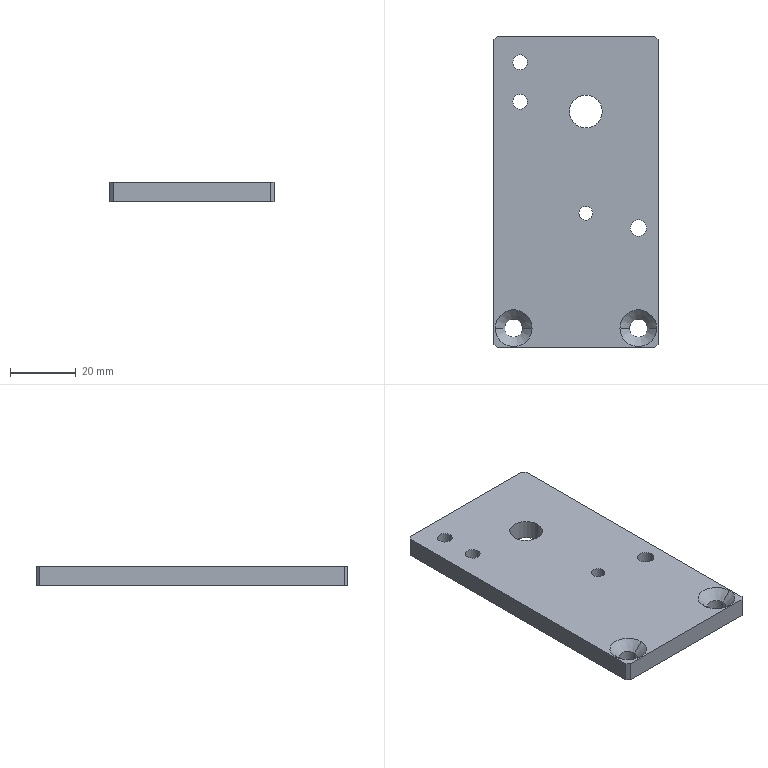Component | SolidWorks | JCT-03-02SmallUprightPlate-1 | 1 solid | 28 faces | box 50 x 95 x 6 mm | volume 27151 mm3 | cylinder 14 | plane 10 | cone 4 | commonest cylinder face diameters 4.5 x4 5.5 x4 10 x2 4.2 x2 5 x2
build123d program:
from build123d import *

# Parameters (mm, degrees)
SKETCH1_W                                            = 50
SKETCH1_H                                            = 95
EXTRUDE1_DEPTH                                       = 3
M5_HEXAGONAL_COUNTERSUNK_SCREW_COUNTERSU_D           = 5.5
M5_HEXAGONAL_COUNTERSUNK_SCREW_COUNTERSU_CSINK_D     = 11.2
M5_HEXAGONAL_COUNTERSUNK_SCREW_COUNTERSU_CSINK_ANGLE = 90
M5_TAPPED_HOLE1_D                                    = 5
M5_TAPPED_HOLE2_D                                    = 4.2
M10_TAPPED_HOLE1_D                                   = 10
SKETCH10_R                                           = 2.25
EXTRUDE2_DEPTH                                       = 108.522
CHAMFER1_SIZE                                        = 1


with BuildPart() as part:
    # Sketch1 → Extrude1 (new, symmetric)
    with BuildSketch(Plane(origin=(0, 0, 0), x_dir=(0, 0, -1), z_dir=(1, 0, 0))):
        with Locations((-25, 47.5)):
            Rectangle(SKETCH1_W, SKETCH1_H)
    extrude(amount=EXTRUDE1_DEPTH, both=True)

    # M5 Hexagonal Countersunk Screw Countersu (through all)
    with Locations(Plane(origin=(3, 0, 0), x_dir=(0, 0, -1), z_dir=(1, 0, 0))):
        with Locations((-44, 6), (-6, 6)):
            CounterSinkHole(M5_HEXAGONAL_COUNTERSUNK_SCREW_COUNTERSU_D / 2, M5_HEXAGONAL_COUNTERSUNK_SCREW_COUNTERSU_CSINK_D / 2, counter_sink_angle=M5_HEXAGONAL_COUNTERSUNK_SCREW_COUNTERSU_CSINK_ANGLE)

    # M5 Tapped Hole1 (through all)
    with Locations(Plane(origin=(3, 0, 0), x_dir=(0, 0, -1), z_dir=(1, 0, 0))):
        with Locations((-6, 36.5)):
            Hole(M5_TAPPED_HOLE1_D / 2)

    # M5 Tapped Hole2 (through all)
    with Locations(Plane(origin=(3, 0, 0), x_dir=(0, 0, -1), z_dir=(1, 0, 0))):
        with Locations((-22, 41)):
            Hole(M5_TAPPED_HOLE2_D / 2)

    # M10 Tapped Hole1 (through all)
    with Locations(Plane(origin=(3, 0, 0), x_dir=(0, 0, -1), z_dir=(1, 0, 0))):
        with Locations((-22, 72)):
            Hole(M10_TAPPED_HOLE1_D / 2)

    # Sketch10 → Extrude2 (cut, through all)
    with BuildSketch(Plane(origin=(3, 0, 0), x_dir=(0, 0, -1), z_dir=(1, 0, 0))):
        with Locations((-42, 87)):
            Circle(SKETCH10_R)
        with Locations((-42, 75)):
            Circle(SKETCH10_R)
    extrude(amount=-EXTRUDE2_DEPTH, mode=Mode.SUBTRACT)

    # Chamfer1
    chamfer1_edges = [part.edges().sort_by_distance(p)[0] for p in [
        (0, 0, 0),
        (0, 0, 50),
        (0, 95, 50),
        (0, 95, 0),
    ]]
    chamfer(chamfer1_edges, length=CHAMFER1_SIZE)


solid = part.part

# Placed as in the assembly
solid = solid.moved(Location((29.266, -2.701, 59), (0, -90, 0)))
STEP:
#1=CARTESIAN_POINT('',(-0.5899,2.846,2.205));
#2=VERTEX_POINT('',#1);
#3=CARTESIAN_POINT('',(-0.4127,2.846,2.205));
#4=VERTEX_POINT('',#3);
#5=CARTESIAN_POINT('',(-0.5013,2.846,2.205));
#6=DIRECTION('',(0.,-0.,1.));
#7=DIRECTION('',(1.,0.,0.));
#8=AXIS2_PLACEMENT_3D('',#5,#6,#7);
#9=CIRCLE('',#8,0.08858);
#10=EDGE_CURVE('',#2,#4,#9,.T.);
#11=ORIENTED_EDGE('',*,*,#10,.F.);
#12=CARTESIAN_POINT('',(-0.5899,2.846,2.441));
#13=VERTEX_POINT('',#12);
#14=CARTESIAN_POINT('',(-0.5899,2.846,2.205));
#15=DIRECTION('',(0.,-0.,1.));
#16=VECTOR('',#15,39.37);
#17=LINE('',#14,#16);
#18=EDGE_CURVE('',#2,#13,#17,.T.);
#19=ORIENTED_EDGE('',*,*,#18,.T.);
#20=CARTESIAN_POINT('',(-0.4127,2.846,2.441));
#21=VERTEX_POINT('',#20);
#22=CARTESIAN_POINT('',(-0.5013,2.846,2.441));
#23=DIRECTION('',(0.,-0.,1.));
#24=DIRECTION('',(1.,0.,0.));
#25=AXIS2_PLACEMENT_3D('',#22,#23,#24);
#26=CIRCLE('',#25,0.08858);
#27=EDGE_CURVE('',#13,#21,#26,.T.);
#28=ORIENTED_EDGE('',*,*,#27,.T.);
#29=CARTESIAN_POINT('',(-0.4127,2.846,2.205));
#30=DIRECTION('',(0.,-0.,1.));
#31=VECTOR('',#30,39.37);
#32=LINE('',#29,#31);
#33=EDGE_CURVE('',#4,#21,#32,.T.);
#34=ORIENTED_EDGE('',*,*,#33,.F.);
#35=EDGE_LOOP('',(#11,#19,#28,#34));
#36=FACE_OUTER_BOUND('',#35,.T.);
#37=CARTESIAN_POINT('',(-0.5013,2.846,2.205));
#38=DIRECTION('',(0.,-0.,1.));
#39=DIRECTION('',(1.,0.,0.));
#40=AXIS2_PLACEMENT_3D('',#37,#38,#39);
#41=CYLINDRICAL_SURFACE('',#40,0.08858);
#42=ADVANCED_FACE('',(#36),#41,.F.);
#43=CARTESIAN_POINT('',(-0.5899,3.319,2.205));
#44=VERTEX_POINT('',#43);
#45=CARTESIAN_POINT('',(-0.4127,3.319,2.205));
#46=VERTEX_POINT('',#45);
#47=CARTESIAN_POINT('',(-0.5013,3.319,2.205));
#48=DIRECTION('',(0.,-0.,1.));
#49=DIRECTION('',(1.,0.,0.));
#50=AXIS2_PLACEMENT_3D('',#47,#48,#49);
#51=CIRCLE('',#50,0.08858);
#52=EDGE_CURVE('',#44,#46,#51,.T.);
#53=ORIENTED_EDGE('',*,*,#52,.F.);
#54=CARTESIAN_POINT('',(-0.5899,3.319,2.441));
#55=VERTEX_POINT('',#54);
#56=CARTESIAN_POINT('',(-0.5899,3.319,2.205));
#57=DIRECTION('',(0.,-0.,1.));
#58=VECTOR('',#57,39.37);
#59=LINE('',#56,#58);
#60=EDGE_CURVE('',#44,#55,#59,.T.);
#61=ORIENTED_EDGE('',*,*,#60,.T.);
#62=CARTESIAN_POINT('',(-0.4127,3.319,2.441));
#63=VERTEX_POINT('',#62);
#64=CARTESIAN_POINT('',(-0.5013,3.319,2.441));
#65=DIRECTION('',(0.,-0.,1.));
#66=DIRECTION('',(1.,0.,0.));
#67=AXIS2_PLACEMENT_3D('',#64,#65,#66);
#68=CIRCLE('',#67,0.08858);
#69=EDGE_CURVE('',#55,#63,#68,.T.);
#70=ORIENTED_EDGE('',*,*,#69,.T.);
#71=CARTESIAN_POINT('',(-0.4127,3.319,2.205));
#72=DIRECTION('',(0.,-0.,1.));
#73=VECTOR('',#72,39.37);
#74=LINE('',#71,#73);
#75=EDGE_CURVE('',#46,#63,#74,.T.);
#76=ORIENTED_EDGE('',*,*,#75,.F.);
#77=EDGE_LOOP('',(#53,#61,#70,#76));
#78=FACE_OUTER_BOUND('',#77,.T.);
#79=CARTESIAN_POINT('',(-0.5013,3.319,2.205));
#80=DIRECTION('',(0.,-0.,1.));
#81=DIRECTION('',(1.,0.,0.));
#82=AXIS2_PLACEMENT_3D('',#79,#80,#81);
#83=CYLINDRICAL_SURFACE('',#82,0.08858);
#84=ADVANCED_FACE('',(#78),#83,.F.);
#85=CARTESIAN_POINT('',(0.08922,2.728,2.205));
#86=VERTEX_POINT('',#85);
#87=CARTESIAN_POINT('',(0.4829,2.728,2.205));
#88=VERTEX_POINT('',#87);
#89=CARTESIAN_POINT('',(0.2861,2.728,2.205));
#90=DIRECTION('',(0.,-0.,1.));
#91=DIRECTION('',(1.,0.,0.));
#92=AXIS2_PLACEMENT_3D('',#89,#90,#91);
#93=CIRCLE('',#92,0.1969);
#94=EDGE_CURVE('',#86,#88,#93,.T.);
#95=ORIENTED_EDGE('',*,*,#94,.F.);
#96=CARTESIAN_POINT('',(0.08922,2.728,2.441));
#97=VERTEX_POINT('',#96);
#98=CARTESIAN_POINT('',(0.08922,2.728,2.441));
#99=DIRECTION('',(0.,-0.,1.));
#100=VECTOR('',#99,39.37);
#101=LINE('',#98,#100);
#102=EDGE_CURVE('',#86,#97,#101,.T.);
#103=ORIENTED_EDGE('',*,*,#102,.T.);
#104=CARTESIAN_POINT('',(0.4829,2.728,2.441));
#105=VERTEX_POINT('',#104);
#106=CARTESIAN_POINT('',(0.2861,2.728,2.441));
#107=DIRECTION('',(0.,-0.,1.));
#108=DIRECTION('',(1.,0.,0.));
#109=AXIS2_PLACEMENT_3D('',#106,#107,#108);
#110=CIRCLE('',#109,0.1969);
#111=EDGE_CURVE('',#97,#105,#110,.T.);
#112=ORIENTED_EDGE('',*,*,#111,.T.);
#113=CARTESIAN_POINT('',(0.4829,2.728,2.441));
#114=DIRECTION('',(0.,-0.,1.));
#115=VECTOR('',#114,39.37);
#116=LINE('',#113,#115);
#117=EDGE_CURVE('',#88,#105,#116,.T.);
#118=ORIENTED_EDGE('',*,*,#117,.F.);
#119=EDGE_LOOP('',(#95,#103,#112,#118));
#120=FACE_OUTER_BOUND('',#119,.T.);
#121=CARTESIAN_POINT('',(0.2861,2.728,2.441));
#122=DIRECTION('',(0.,-0.,1.));
#123=DIRECTION('',(1.,0.,0.));
#124=AXIS2_PLACEMENT_3D('',#121,#122,#123);
#125=CYLINDRICAL_SURFACE('',#124,0.1969);
#126=ADVANCED_FACE('',(#120),#125,.F.);
#127=CARTESIAN_POINT('',(0.2034,1.508,2.205));
#128=VERTEX_POINT('',#127);
#129=CARTESIAN_POINT('',(0.3688,1.508,2.205));
#130=VERTEX_POINT('',#129);
#131=CARTESIAN_POINT('',(0.2861,1.508,2.205));
#132=DIRECTION('',(0.,-0.,1.));
#133=DIRECTION('',(1.,0.,0.));
#134=AXIS2_PLACEMENT_3D('',#131,#132,#133);
#135=CIRCLE('',#134,0.08268);
#136=EDGE_CURVE('',#128,#130,#135,.T.);
#137=ORIENTED_EDGE('',*,*,#136,.F.);
#138=CARTESIAN_POINT('',(0.2034,1.508,2.441));
#139=VERTEX_POINT('',#138);
#140=CARTESIAN_POINT('',(0.2034,1.508,2.441));
#141=DIRECTION('',(0.,-0.,1.));
#142=VECTOR('',#141,39.37);
#143=LINE('',#140,#142);
#144=EDGE_CURVE('',#128,#139,#143,.T.);
#145=ORIENTED_EDGE('',*,*,#144,.T.);
#146=CARTESIAN_POINT('',(0.3688,1.508,2.441));
#147=VERTEX_POINT('',#146);
#148=CARTESIAN_POINT('',(0.2861,1.508,2.441));
#149=DIRECTION('',(0.,-0.,1.));
#150=DIRECTION('',(1.,0.,0.));
#151=AXIS2_PLACEMENT_3D('',#148,#149,#150);
#152=CIRCLE('',#151,0.08268);
#153=EDGE_CURVE('',#139,#147,#152,.T.);
#154=ORIENTED_EDGE('',*,*,#153,.T.);
#155=CARTESIAN_POINT('',(0.3688,1.508,2.441));
#156=DIRECTION('',(0.,-0.,1.));
#157=VECTOR('',#156,39.37);
#158=LINE('',#155,#157);
#159=EDGE_CURVE('',#130,#147,#158,.T.);
#160=ORIENTED_EDGE('',*,*,#159,.F.);
#161=EDGE_LOOP('',(#137,#145,#154,#160));
#162=FACE_OUTER_BOUND('',#161,.T.);
#163=CARTESIAN_POINT('',(0.2861,1.508,2.441));
#164=DIRECTION('',(0.,-0.,1.));
#165=DIRECTION('',(1.,0.,0.));
#166=AXIS2_PLACEMENT_3D('',#163,#164,#165);
#167=CYLINDRICAL_SURFACE('',#166,0.08268);
#168=ADVANCED_FACE('',(#162),#167,.F.);
#169=CARTESIAN_POINT('',(0.8176,1.331,2.205));
#170=VERTEX_POINT('',#169);
#171=CARTESIAN_POINT('',(1.014,1.331,2.205));
#172=VERTEX_POINT('',#171);
#173=CARTESIAN_POINT('',(0.916,1.331,2.205));
#174=DIRECTION('',(0.,-0.,1.));
#175=DIRECTION('',(1.,0.,0.));
#176=AXIS2_PLACEMENT_3D('',#173,#174,#175);
#177=CIRCLE('',#176,0.09843);
#178=EDGE_CURVE('',#170,#172,#177,.T.);
#179=ORIENTED_EDGE('',*,*,#178,.F.);
#180=CARTESIAN_POINT('',(0.8176,1.331,2.441));
#181=VERTEX_POINT('',#180);
#182=CARTESIAN_POINT('',(0.8176,1.331,2.441));
#183=DIRECTION('',(0.,-0.,1.));
#184=VECTOR('',#183,39.37);
#185=LINE('',#182,#184);
#186=EDGE_CURVE('',#170,#181,#185,.T.);
#187=ORIENTED_EDGE('',*,*,#186,.T.);
#188=CARTESIAN_POINT('',(1.014,1.331,2.441));
#189=VERTEX_POINT('',#188);
#190=CARTESIAN_POINT('',(0.916,1.331,2.441));
#191=DIRECTION('',(0.,-0.,1.));
#192=DIRECTION('',(1.,0.,0.));
#193=AXIS2_PLACEMENT_3D('',#190,#191,#192);
#194=CIRCLE('',#193,0.09843);
#195=EDGE_CURVE('',#181,#189,#194,.T.);
#196=ORIENTED_EDGE('',*,*,#195,.T.);
#197=CARTESIAN_POINT('',(1.014,1.331,2.441));
#198=DIRECTION('',(0.,-0.,1.));
#199=VECTOR('',#198,39.37);
#200=LINE('',#197,#199);
#201=EDGE_CURVE('',#172,#189,#200,.T.);
#202=ORIENTED_EDGE('',*,*,#201,.F.);
#203=EDGE_LOOP('',(#179,#187,#196,#202));
#204=FACE_OUTER_BOUND('',#203,.T.);
#205=CARTESIAN_POINT('',(0.916,1.331,2.441));
#206=DIRECTION('',(0.,-0.,1.));
#207=DIRECTION('',(1.,0.,0.));
#208=AXIS2_PLACEMENT_3D('',#205,#206,#207);
#209=CYLINDRICAL_SURFACE('',#208,0.09843);
#210=ADVANCED_FACE('',(#204),#209,.F.);
#211=CARTESIAN_POINT('',(-0.6883,0.1299,2.329));
#212=VERTEX_POINT('',#211);
#213=CARTESIAN_POINT('',(-0.4718,0.1299,2.329));
#214=VERTEX_POINT('',#213);
#215=CARTESIAN_POINT('',(-0.5801,0.1299,2.329));
#216=DIRECTION('',(0.,-0.,1.));
#217=DIRECTION('',(1.,-0.,0.));
#218=AXIS2_PLACEMENT_3D('',#215,#216,#217);
#219=CIRCLE('',#218,0.1083);
#220=EDGE_CURVE('',#212,#214,#219,.T.);
#221=ORIENTED_EDGE('',*,*,#220,.F.);
#222=CARTESIAN_POINT('',(-0.8005,0.1299,2.441));
#223=VERTEX_POINT('',#222);
#224=CARTESIAN_POINT('',(-0.8005,0.1299,2.441));
#225=DIRECTION('',(-0.7071,0.,0.7071));
#226=VECTOR('',#225,39.37);
#227=LINE('',#224,#226);
#228=EDGE_CURVE('',#212,#223,#227,.T.);
#229=ORIENTED_EDGE('',*,*,#228,.T.);
#230=CARTESIAN_POINT('',(-0.3596,0.1299,2.441));
#231=VERTEX_POINT('',#230);
#232=CARTESIAN_POINT('',(-0.5801,0.1299,2.441));
#233=DIRECTION('',(0.,-0.,1.));
#234=DIRECTION('',(1.,-0.,0.));
#235=AXIS2_PLACEMENT_3D('',#232,#233,#234);
#236=CIRCLE('',#235,0.2205);
#237=EDGE_CURVE('',#223,#231,#236,.T.);
#238=ORIENTED_EDGE('',*,*,#237,.T.);
#239=CARTESIAN_POINT('',(-0.3596,0.1299,2.441));
#240=DIRECTION('',(0.7071,-0.,0.7071));
#241=VECTOR('',#240,39.37);
#242=LINE('',#239,#241);
#243=EDGE_CURVE('',#214,#231,#242,.T.);
#244=ORIENTED_EDGE('',*,*,#243,.F.);
#245=EDGE_LOOP('',(#221,#229,#238,#244));
#246=FACE_OUTER_BOUND('',#245,.T.);
#247=CARTESIAN_POINT('',(-0.5801,0.1299,2.441));
#248=DIRECTION('',(0.,-0.,1.));
#249=DIRECTION('',(1.,-0.,0.));
#250=AXIS2_PLACEMENT_3D('',#247,#248,#249);
#251=CONICAL_SURFACE('',#250,0.2205,0.7854);
#252=ADVANCED_FACE('',(#246),#251,.F.);
#253=CARTESIAN_POINT('',(-0.6883,0.1299,2.205));
#254=VERTEX_POINT('',#253);
#255=CARTESIAN_POINT('',(-0.4718,0.1299,2.205));
#256=VERTEX_POINT('',#255);
#257=CARTESIAN_POINT('',(-0.5801,0.1299,2.205));
#258=DIRECTION('',(0.,-0.,1.));
#259=DIRECTION('',(1.,-0.,0.));
#260=AXIS2_PLACEMENT_3D('',#257,#258,#259);
#261=CIRCLE('',#260,0.1083);
#262=EDGE_CURVE('',#254,#256,#261,.T.);
#263=ORIENTED_EDGE('',*,*,#262,.F.);
#264=CARTESIAN_POINT('',(-0.6883,0.1299,2.441));
#265=DIRECTION('',(0.,-0.,1.));
#266=VECTOR('',#265,39.37);
#267=LINE('',#264,#266);
#268=EDGE_CURVE('',#254,#212,#267,.T.);
#269=ORIENTED_EDGE('',*,*,#268,.T.);
#270=ORIENTED_EDGE('',*,*,#220,.T.);
#271=CARTESIAN_POINT('',(-0.4718,0.1299,2.441));
#272=DIRECTION('',(0.,-0.,1.));
#273=VECTOR('',#272,39.37);
#274=LINE('',#271,#273);
#275=EDGE_CURVE('',#256,#214,#274,.T.);
#276=ORIENTED_EDGE('',*,*,#275,.F.);
#277=EDGE_LOOP('',(#263,#269,#270,#276));
#278=FACE_OUTER_BOUND('',#277,.T.);
#279=CARTESIAN_POINT('',(-0.5801,0.1299,2.441));
#280=DIRECTION('',(0.,-0.,1.));
#281=DIRECTION('',(1.,-0.,0.));
#282=AXIS2_PLACEMENT_3D('',#279,#280,#281);
#283=CYLINDRICAL_SURFACE('',#282,0.1083);
#284=ADVANCED_FACE('',(#278),#283,.F.);
#285=CARTESIAN_POINT('',(0.8077,0.1299,2.329));
#286=VERTEX_POINT('',#285);
#287=CARTESIAN_POINT('',(1.024,0.1299,2.329));
#288=VERTEX_POINT('',#287);
#289=CARTESIAN_POINT('',(0.916,0.1299,2.329));
#290=DIRECTION('',(0.,-0.,1.));
#291=DIRECTION('',(1.,-0.,0.));
#292=AXIS2_PLACEMENT_3D('',#289,#290,#291);
#293=CIRCLE('',#292,0.1083);
#294=EDGE_CURVE('',#286,#288,#293,.T.);
#295=ORIENTED_EDGE('',*,*,#294,.F.);
#296=CARTESIAN_POINT('',(0.6955,0.1299,2.441));
#297=VERTEX_POINT('',#296);
#298=CARTESIAN_POINT('',(0.6955,0.1299,2.441));
#299=DIRECTION('',(-0.7071,0.,0.7071));
#300=VECTOR('',#299,39.37);
#301=LINE('',#298,#300);
#302=EDGE_CURVE('',#286,#297,#301,.T.);
#303=ORIENTED_EDGE('',*,*,#302,.T.);
#304=CARTESIAN_POINT('',(1.136,0.1299,2.441));
#305=VERTEX_POINT('',#304);
#306=CARTESIAN_POINT('',(0.916,0.1299,2.441));
#307=DIRECTION('',(0.,-0.,1.));
#308=DIRECTION('',(1.,-0.,0.));
#309=AXIS2_PLACEMENT_3D('',#306,#307,#308);
#310=CIRCLE('',#309,0.2205);
#311=EDGE_CURVE('',#297,#305,#310,.T.);
#312=ORIENTED_EDGE('',*,*,#311,.T.);
#313=CARTESIAN_POINT('',(1.136,0.1299,2.441));
#314=DIRECTION('',(0.7071,-0.,0.7071));
#315=VECTOR('',#314,39.37);
#316=LINE('',#313,#315);
#317=EDGE_CURVE('',#288,#305,#316,.T.);
#318=ORIENTED_EDGE('',*,*,#317,.F.);
#319=EDGE_LOOP('',(#295,#303,#312,#318));
#320=FACE_OUTER_BOUND('',#319,.T.);
#321=CARTESIAN_POINT('',(0.916,0.1299,2.441));
#322=DIRECTION('',(0.,-0.,1.));
#323=DIRECTION('',(1.,-0.,0.));
#324=AXIS2_PLACEMENT_3D('',#321,#322,#323);
#325=CONICAL_SURFACE('',#324,0.2205,0.7854);
#326=ADVANCED_FACE('',(#320),#325,.F.);
#327=CARTESIAN_POINT('',(0.8077,0.1299,2.205));
#328=VERTEX_POINT('',#327);
#329=CARTESIAN_POINT('',(1.024,0.1299,2.205));
#330=VERTEX_POINT('',#329);
#331=CARTESIAN_POINT('',(0.916,0.1299,2.205));
#332=DIRECTION('',(0.,-0.,1.));
#333=DIRECTION('',(1.,-0.,0.));
#334=AXIS2_PLACEMENT_3D('',#331,#332,#333);
#335=CIRCLE('',#334,0.1083);
#336=EDGE_CURVE('',#328,#330,#335,.T.);
#337=ORIENTED_EDGE('',*,*,#336,.F.);
#338=CARTESIAN_POINT('',(0.8077,0.1299,2.441));
#339=DIRECTION('',(0.,-0.,1.));
#340=VECTOR('',#339,39.37);
#341=LINE('',#338,#340);
#342=EDGE_CURVE('',#328,#286,#341,.T.);
#343=ORIENTED_EDGE('',*,*,#342,.T.);
#344=ORIENTED_EDGE('',*,*,#294,.T.);
#345=CARTESIAN_POINT('',(1.024,0.1299,2.441));
#346=DIRECTION('',(0.,-0.,1.));
#347=VECTOR('',#346,39.37);
#348=LINE('',#345,#347);
#349=EDGE_CURVE('',#330,#288,#348,.T.);
#350=ORIENTED_EDGE('',*,*,#349,.F.);
#351=EDGE_LOOP('',(#337,#343,#344,#350));
#352=FACE_OUTER_BOUND('',#351,.T.);
#353=CARTESIAN_POINT('',(0.916,0.1299,2.441));
#354=DIRECTION('',(0.,-0.,1.));
#355=DIRECTION('',(1.,-0.,0.));
#356=AXIS2_PLACEMENT_3D('',#353,#354,#355);
#357=CYLINDRICAL_SURFACE('',#356,0.1083);
#358=ADVANCED_FACE('',(#352),#357,.F.);
#359=CARTESIAN_POINT('',(1.152,-0.06696,2.441));
#360=VERTEX_POINT('',#359);
#361=CARTESIAN_POINT('',(1.152,3.594,2.441));
#362=VERTEX_POINT('',#361);
#363=CARTESIAN_POINT('',(1.152,-0.1063,2.441));
#364=DIRECTION('',(0.,1.,0.));
#365=VECTOR('',#364,39.37);
#366=LINE('',#363,#365);
#367=EDGE_CURVE('',#360,#362,#366,.T.);
#368=ORIENTED_EDGE('',*,*,#367,.F.);
#369=CARTESIAN_POINT('',(1.152,-0.06696,2.205));
#370=VERTEX_POINT('',#369);
#371=CARTESIAN_POINT('',(1.152,-0.06696,2.441));
#372=DIRECTION('',(-0.,0.,-1.));
#373=VECTOR('',#372,39.37);
#374=LINE('',#371,#373);
#375=EDGE_CURVE('',#360,#370,#374,.T.);
#376=ORIENTED_EDGE('',*,*,#375,.T.);
#377=CARTESIAN_POINT('',(1.152,3.594,2.205));
#378=VERTEX_POINT('',#377);
#379=CARTESIAN_POINT('',(1.152,-0.1063,2.205));
#380=DIRECTION('',(0.,1.,0.));
#381=VECTOR('',#380,39.37);
#382=LINE('',#379,#381);
#383=EDGE_CURVE('',#370,#378,#382,.T.);
#384=ORIENTED_EDGE('',*,*,#383,.T.);
#385=CARTESIAN_POINT('',(1.152,3.594,2.441));
#386=DIRECTION('',(0.,-0.,1.));
#387=VECTOR('',#386,39.37);
#388=LINE('',#385,#387);
#389=EDGE_CURVE('',#378,#362,#388,.T.);
#390=ORIENTED_EDGE('',*,*,#389,.T.);
#391=EDGE_LOOP('',(#368,#376,#384,#390));
#392=FACE_OUTER_BOUND('',#391,.T.);
#393=CARTESIAN_POINT('',(1.152,-0.1063,2.441));
#394=DIRECTION('',(-1.,0.,0.));
#395=DIRECTION('',(0.,-0.,1.));
#396=AXIS2_PLACEMENT_3D('',#393,#394,#395);
#397=PLANE('',#396);
#398=ADVANCED_FACE('',(#392),#397,.F.);
#399=CARTESIAN_POINT('',(1.113,3.634,2.441));
#400=VERTEX_POINT('',#399);
#401=CARTESIAN_POINT('',(-0.7769,3.634,2.441));
#402=VERTEX_POINT('',#401);
#403=CARTESIAN_POINT('',(1.152,3.634,2.441));
#404=DIRECTION('',(-1.,0.,0.));
#405=VECTOR('',#404,39.37);
#406=LINE('',#403,#405);
#407=EDGE_CURVE('',#400,#402,#406,.T.);
#408=ORIENTED_EDGE('',*,*,#407,.F.);
#409=CARTESIAN_POINT('',(1.113,3.634,2.205));
#410=VERTEX_POINT('',#409);
#411=CARTESIAN_POINT('',(1.113,3.634,2.441));
#412=DIRECTION('',(-0.,0.,-1.));
#413=VECTOR('',#412,39.37);
#414=LINE('',#411,#413);
#415=EDGE_CURVE('',#400,#410,#414,.T.);
#416=ORIENTED_EDGE('',*,*,#415,.T.);
#417=CARTESIAN_POINT('',(-0.7769,3.634,2.205));
#418=VERTEX_POINT('',#417);
#419=CARTESIAN_POINT('',(1.152,3.634,2.205));
#420=DIRECTION('',(-1.,0.,0.));
#421=VECTOR('',#420,39.37);
#422=LINE('',#419,#421);
#423=EDGE_CURVE('',#410,#418,#422,.T.);
#424=ORIENTED_EDGE('',*,*,#423,.T.);
#425=CARTESIAN_POINT('',(-0.7769,3.634,2.441));
#426=DIRECTION('',(0.,-0.,1.));
#427=VECTOR('',#426,39.37);
#428=LINE('',#425,#427);
#429=EDGE_CURVE('',#418,#402,#428,.T.);
#430=ORIENTED_EDGE('',*,*,#429,.T.);
#431=EDGE_LOOP('',(#408,#416,#424,#430));
#432=FACE_OUTER_BOUND('',#431,.T.);
#433=CARTESIAN_POINT('',(1.152,3.634,2.441));
#434=DIRECTION('',(-0.,-1.,-0.));
#435=DIRECTION('',(1.,-0.,-0.));
#436=AXIS2_PLACEMENT_3D('',#433,#434,#435);
#437=PLANE('',#436);
#438=ADVANCED_FACE('',(#432),#437,.F.);
#439=CARTESIAN_POINT('',(-0.8163,3.594,2.205));
#440=VERTEX_POINT('',#439);
#441=CARTESIAN_POINT('',(-0.8163,-0.06696,2.205));
#442=VERTEX_POINT('',#441);
#443=CARTESIAN_POINT('',(-0.8163,-0.1063,2.205));
#444=DIRECTION('',(-0.,-1.,-0.));
#445=VECTOR('',#444,39.37);
#446=LINE('',#443,#445);
#447=EDGE_CURVE('',#440,#442,#446,.T.);
#448=ORIENTED_EDGE('',*,*,#447,.T.);
#449=CARTESIAN_POINT('',(-0.8163,-0.06696,2.441));
#450=VERTEX_POINT('',#449);
#451=CARTESIAN_POINT('',(-0.8163,-0.06696,2.441));
#452=DIRECTION('',(0.,-0.,1.));
#453=VECTOR('',#452,39.37);
#454=LINE('',#451,#453);
#455=EDGE_CURVE('',#442,#450,#454,.T.);
#456=ORIENTED_EDGE('',*,*,#455,.T.);
#457=CARTESIAN_POINT('',(-0.8163,3.594,2.441));
#458=VERTEX_POINT('',#457);
#459=CARTESIAN_POINT('',(-0.8163,-0.1063,2.441));
#460=DIRECTION('',(-0.,-1.,-0.));
#461=VECTOR('',#460,39.37);
#462=LINE('',#459,#461);
#463=EDGE_CURVE('',#458,#450,#462,.T.);
#464=ORIENTED_EDGE('',*,*,#463,.F.);
#465=CARTESIAN_POINT('',(-0.8163,3.594,2.441));
#466=DIRECTION('',(-0.,0.,-1.));
#467=VECTOR('',#466,39.37);
#468=LINE('',#465,#467);
#469=EDGE_CURVE('',#458,#440,#468,.T.);
#470=ORIENTED_EDGE('',*,*,#469,.T.);
#471=EDGE_LOOP('',(#448,#456,#464,#470));
#472=FACE_OUTER_BOUND('',#471,.T.);
#473=CARTESIAN_POINT('',(-0.8163,-0.1063,2.441));
#474=DIRECTION('',(1.,-0.,-0.));
#475=DIRECTION('',(-0.,0.,-1.));
#476=AXIS2_PLACEMENT_3D('',#473,#474,#475);
#477=PLANE('',#476);
#478=ADVANCED_FACE('',(#472),#477,.F.);
#479=CARTESIAN_POINT('',(-0.7769,-0.1063,2.441));
#480=VERTEX_POINT('',#479);
#481=CARTESIAN_POINT('',(1.113,-0.1063,2.441));
#482=VERTEX_POINT('',#481);
#483=CARTESIAN_POINT('',(1.152,-0.1063,2.441));
#484=DIRECTION('',(1.,-0.,-0.));
#485=VECTOR('',#484,39.37);
#486=LINE('',#483,#485);
#487=EDGE_CURVE('',#480,#482,#486,.T.);
#488=ORIENTED_EDGE('',*,*,#487,.F.);
#489=CARTESIAN_POINT('',(-0.7769,-0.1063,2.205));
#490=VERTEX_POINT('',#489);
#491=CARTESIAN_POINT('',(-0.7769,-0.1063,2.441));
#492=DIRECTION('',(-0.,0.,-1.));
#493=VECTOR('',#492,39.37);
#494=LINE('',#491,#493);
#495=EDGE_CURVE('',#480,#490,#494,.T.);
#496=ORIENTED_EDGE('',*,*,#495,.T.);
#497=CARTESIAN_POINT('',(1.113,-0.1063,2.205));
#498=VERTEX_POINT('',#497);
#499=CARTESIAN_POINT('',(1.152,-0.1063,2.205));
#500=DIRECTION('',(1.,-0.,-0.));
#501=VECTOR('',#500,39.37);
#502=LINE('',#499,#501);
#503=EDGE_CURVE('',#490,#498,#502,.T.);
#504=ORIENTED_EDGE('',*,*,#503,.T.);
#505=CARTESIAN_POINT('',(1.113,-0.1063,2.441));
#506=DIRECTION('',(0.,-0.,1.));
#507=VECTOR('',#506,39.37);
#508=LINE('',#505,#507);
#509=EDGE_CURVE('',#498,#482,#508,.T.);
#510=ORIENTED_EDGE('',*,*,#509,.T.);
#511=EDGE_LOOP('',(#488,#496,#504,#510));
#512=FACE_OUTER_BOUND('',#511,.T.);
#513=CARTESIAN_POINT('',(1.152,-0.1063,2.441));
#514=DIRECTION('',(0.,1.,0.));
#515=DIRECTION('',(-1.,0.,0.));
#516=AXIS2_PLACEMENT_3D('',#513,#514,#515);
#517=PLANE('',#516);
#518=ADVANCED_FACE('',(#512),#517,.F.);
#519=CARTESIAN_POINT('',(-0.5013,2.846,2.441));
#520=DIRECTION('',(0.,-0.,1.));
#521=DIRECTION('',(1.,0.,0.));
#522=AXIS2_PLACEMENT_3D('',#519,#520,#521);
#523=CIRCLE('',#522,0.08858);
#524=EDGE_CURVE('',#21,#13,#523,.T.);
#525=ORIENTED_EDGE('',*,*,#524,.F.);
#526=ORIENTED_EDGE('',*,*,#27,.F.);
#527=EDGE_LOOP('',(#525,#526));
#528=FACE_BOUND('',#527,.T.);
#529=CARTESIAN_POINT('',(-0.5013,3.319,2.441));
#530=DIRECTION('',(0.,-0.,1.));
#531=DIRECTION('',(1.,0.,0.));
#532=AXIS2_PLACEMENT_3D('',#529,#530,#531);
#533=CIRCLE('',#532,0.08858);
#534=EDGE_CURVE('',#63,#55,#533,.T.);
#535=ORIENTED_EDGE('',*,*,#534,.F.);
#536=ORIENTED_EDGE('',*,*,#69,.F.);
#537=EDGE_LOOP('',(#535,#536));
#538=FACE_BOUND('',#537,.T.);
#539=CARTESIAN_POINT('',(0.2861,2.728,2.441));
#540=DIRECTION('',(0.,-0.,1.));
#541=DIRECTION('',(1.,0.,0.));
#542=AXIS2_PLACEMENT_3D('',#539,#540,#541);
#543=CIRCLE('',#542,0.1969);
#544=EDGE_CURVE('',#105,#97,#543,.T.);
#545=ORIENTED_EDGE('',*,*,#544,.F.);
#546=ORIENTED_EDGE('',*,*,#111,.F.);
#547=EDGE_LOOP('',(#545,#546));
#548=FACE_BOUND('',#547,.T.);
#549=CARTESIAN_POINT('',(0.2861,1.508,2.441));
#550=DIRECTION('',(0.,-0.,1.));
#551=DIRECTION('',(1.,0.,0.));
#552=AXIS2_PLACEMENT_3D('',#549,#550,#551);
#553=CIRCLE('',#552,0.08268);
#554=EDGE_CURVE('',#147,#139,#553,.T.);
#555=ORIENTED_EDGE('',*,*,#554,.F.);
#556=ORIENTED_EDGE('',*,*,#153,.F.);
#557=EDGE_LOOP('',(#555,#556));
#558=FACE_BOUND('',#557,.T.);
#559=CARTESIAN_POINT('',(0.916,1.331,2.441));
#560=DIRECTION('',(0.,-0.,1.));
#561=DIRECTION('',(1.,0.,0.));
#562=AXIS2_PLACEMENT_3D('',#559,#560,#561);
#563=CIRCLE('',#562,0.09843);
#564=EDGE_CURVE('',#189,#181,#563,.T.);
#565=ORIENTED_EDGE('',*,*,#564,.F.);
#566=ORIENTED_EDGE('',*,*,#195,.F.);
#567=EDGE_LOOP('',(#565,#566));
#568=FACE_BOUND('',#567,.T.);
#569=CARTESIAN_POINT('',(-0.5801,0.1299,2.441));
#570=DIRECTION('',(0.,-0.,1.));
#571=DIRECTION('',(1.,-0.,0.));
#572=AXIS2_PLACEMENT_3D('',#569,#570,#571);
#573=CIRCLE('',#572,0.2205);
#574=EDGE_CURVE('',#231,#223,#573,.T.);
#575=ORIENTED_EDGE('',*,*,#574,.F.);
#576=ORIENTED_EDGE('',*,*,#237,.F.);
#577=EDGE_LOOP('',(#575,#576));
#578=FACE_BOUND('',#577,.T.);
#579=CARTESIAN_POINT('',(0.916,0.1299,2.441));
#580=DIRECTION('',(0.,-0.,1.));
#581=DIRECTION('',(1.,-0.,0.));
#582=AXIS2_PLACEMENT_3D('',#579,#580,#581);
#583=CIRCLE('',#582,0.2205);
#584=EDGE_CURVE('',#305,#297,#583,.T.);
#585=ORIENTED_EDGE('',*,*,#584,.F.);
#586=ORIENTED_EDGE('',*,*,#311,.F.);
#587=EDGE_LOOP('',(#585,#586));
#588=FACE_BOUND('',#587,.T.);
#589=ORIENTED_EDGE('',*,*,#463,.T.);
#590=CARTESIAN_POINT('',(-1.682,0.7992,2.441));
#591=DIRECTION('',(0.7071,-0.7071,-0.));
#592=VECTOR('',#591,39.37);
#593=LINE('',#590,#592);
#594=EDGE_CURVE('',#450,#480,#593,.T.);
#595=ORIENTED_EDGE('',*,*,#594,.T.);
#596=ORIENTED_EDGE('',*,*,#487,.T.);
#597=CARTESIAN_POINT('',(3.003,1.783,2.441));
#598=DIRECTION('',(0.7071,0.7071,0.));
#599=VECTOR('',#598,39.37);
#600=LINE('',#597,#599);
#601=EDGE_CURVE('',#482,#360,#600,.T.);
#602=ORIENTED_EDGE('',*,*,#601,.T.);
#603=ORIENTED_EDGE('',*,*,#367,.T.);
#604=CARTESIAN_POINT('',(1.133,3.614,2.441));
#605=DIRECTION('',(-0.7071,0.7071,0.));
#606=VECTOR('',#605,39.37);
#607=LINE('',#604,#606);
#608=EDGE_CURVE('',#362,#400,#607,.T.);
#609=ORIENTED_EDGE('',*,*,#608,.T.);
#610=ORIENTED_EDGE('',*,*,#407,.T.);
#611=CARTESIAN_POINT('',(0.1876,4.598,2.441));
#612=DIRECTION('',(-0.7071,-0.7071,-0.));
#613=VECTOR('',#612,39.37);
#614=LINE('',#611,#613);
#615=EDGE_CURVE('',#402,#458,#614,.T.);
#616=ORIENTED_EDGE('',*,*,#615,.T.);
#617=EDGE_LOOP('',(#589,#595,#596,#602,#603,#609,#610,#616));
#618=FACE_OUTER_BOUND('',#617,.T.);
#619=CARTESIAN_POINT('',(1.152,3.634,2.441));
#620=DIRECTION('',(0.,-0.,1.));
#621=DIRECTION('',(1.,-0.,-0.));
#622=AXIS2_PLACEMENT_3D('',#619,#620,#621);
#623=PLANE('',#622);
#624=ADVANCED_FACE('',(#528,#538,#548,#558,#568,#578,#588,#618),#623,.T.);
#625=CARTESIAN_POINT('',(-0.5013,2.846,2.205));
#626=DIRECTION('',(0.,-0.,1.));
#627=DIRECTION('',(1.,0.,0.));
#628=AXIS2_PLACEMENT_3D('',#625,#626,#627);
#629=CIRCLE('',#628,0.08858);
#630=EDGE_CURVE('',#4,#2,#629,.T.);
#631=ORIENTED_EDGE('',*,*,#630,.T.);
#632=ORIENTED_EDGE('',*,*,#10,.T.);
#633=EDGE_LOOP('',(#631,#632));
#634=FACE_BOUND('',#633,.T.);
#635=CARTESIAN_POINT('',(-0.5013,3.319,2.205));
#636=DIRECTION('',(0.,-0.,1.));
#637=DIRECTION('',(1.,0.,0.));
#638=AXIS2_PLACEMENT_3D('',#635,#636,#637);
#639=CIRCLE('',#638,0.08858);
#640=EDGE_CURVE('',#46,#44,#639,.T.);
#641=ORIENTED_EDGE('',*,*,#640,.T.);
#642=ORIENTED_EDGE('',*,*,#52,.T.);
#643=EDGE_LOOP('',(#641,#642));
#644=FACE_BOUND('',#643,.T.);
#645=CARTESIAN_POINT('',(0.2861,2.728,2.205));
#646=DIRECTION('',(0.,-0.,1.));
#647=DIRECTION('',(1.,0.,0.));
#648=AXIS2_PLACEMENT_3D('',#645,#646,#647);
#649=CIRCLE('',#648,0.1969);
#650=EDGE_CURVE('',#88,#86,#649,.T.);
#651=ORIENTED_EDGE('',*,*,#650,.T.);
#652=ORIENTED_EDGE('',*,*,#94,.T.);
#653=EDGE_LOOP('',(#651,#652));
#654=FACE_BOUND('',#653,.T.);
#655=CARTESIAN_POINT('',(0.2861,1.508,2.205));
#656=DIRECTION('',(0.,-0.,1.));
#657=DIRECTION('',(1.,0.,0.));
#658=AXIS2_PLACEMENT_3D('',#655,#656,#657);
#659=CIRCLE('',#658,0.08268);
#660=EDGE_CURVE('',#130,#128,#659,.T.);
#661=ORIENTED_EDGE('',*,*,#660,.T.);
#662=ORIENTED_EDGE('',*,*,#136,.T.);
#663=EDGE_LOOP('',(#661,#662));
#664=FACE_BOUND('',#663,.T.);
#665=CARTESIAN_POINT('',(0.916,1.331,2.205));
#666=DIRECTION('',(0.,-0.,1.));
#667=DIRECTION('',(1.,0.,0.));
#668=AXIS2_PLACEMENT_3D('',#665,#666,#667);
#669=CIRCLE('',#668,0.09843);
#670=EDGE_CURVE('',#172,#170,#669,.T.);
#671=ORIENTED_EDGE('',*,*,#670,.T.);
#672=ORIENTED_EDGE('',*,*,#178,.T.);
#673=EDGE_LOOP('',(#671,#672));
#674=FACE_BOUND('',#673,.T.);
#675=CARTESIAN_POINT('',(-0.5801,0.1299,2.205));
#676=DIRECTION('',(0.,-0.,1.));
#677=DIRECTION('',(1.,-0.,0.));
#678=AXIS2_PLACEMENT_3D('',#675,#676,#677);
#679=CIRCLE('',#678,0.1083);
#680=EDGE_CURVE('',#256,#254,#679,.T.);
#681=ORIENTED_EDGE('',*,*,#680,.T.);
#682=ORIENTED_EDGE('',*,*,#262,.T.);
#683=EDGE_LOOP('',(#681,#682));
#684=FACE_BOUND('',#683,.T.);
#685=CARTESIAN_POINT('',(0.916,0.1299,2.205));
#686=DIRECTION('',(0.,-0.,1.));
#687=DIRECTION('',(1.,-0.,0.));
#688=AXIS2_PLACEMENT_3D('',#685,#686,#687);
#689=CIRCLE('',#688,0.1083);
#690=EDGE_CURVE('',#330,#328,#689,.T.);
#691=ORIENTED_EDGE('',*,*,#690,.T.);
#692=ORIENTED_EDGE('',*,*,#336,.T.);
#693=EDGE_LOOP('',(#691,#692));
#694=FACE_BOUND('',#693,.T.);
#695=ORIENTED_EDGE('',*,*,#503,.F.);
#696=CARTESIAN_POINT('',(-0.7769,-0.1063,2.205));
#697=DIRECTION('',(-0.7071,0.7071,0.));
#698=VECTOR('',#697,39.37);
#699=LINE('',#696,#698);
#700=EDGE_CURVE('',#490,#442,#699,.T.);
#701=ORIENTED_EDGE('',*,*,#700,.T.);
#702=ORIENTED_EDGE('',*,*,#447,.F.);
#703=CARTESIAN_POINT('',(-0.8163,3.594,2.205));
#704=DIRECTION('',(0.7071,0.7071,0.));
#705=VECTOR('',#704,39.37);
#706=LINE('',#703,#705);
#707=EDGE_CURVE('',#440,#418,#706,.T.);
#708=ORIENTED_EDGE('',*,*,#707,.T.);
#709=ORIENTED_EDGE('',*,*,#423,.F.);
#710=CARTESIAN_POINT('',(1.113,3.634,2.205));
#711=DIRECTION('',(0.7071,-0.7071,-0.));
#712=VECTOR('',#711,39.37);
#713=LINE('',#710,#712);
#714=EDGE_CURVE('',#410,#378,#713,.T.);
#715=ORIENTED_EDGE('',*,*,#714,.T.);
#716=ORIENTED_EDGE('',*,*,#383,.F.);
#717=CARTESIAN_POINT('',(1.152,-0.06696,2.205));
#718=DIRECTION('',(-0.7071,-0.7071,-0.));
#719=VECTOR('',#718,39.37);
#720=LINE('',#717,#719);
#721=EDGE_CURVE('',#370,#498,#720,.T.);
#722=ORIENTED_EDGE('',*,*,#721,.T.);
#723=EDGE_LOOP('',(#695,#701,#702,#708,#709,#715,#716,#722));
#724=FACE_OUTER_BOUND('',#723,.T.);
#725=CARTESIAN_POINT('',(1.152,3.634,2.205));
#726=DIRECTION('',(0.,-0.,1.));
#727=DIRECTION('',(1.,-0.,-0.));
#728=AXIS2_PLACEMENT_3D('',#725,#726,#727);
#729=PLANE('',#728);
#730=ADVANCED_FACE('',(#634,#644,#654,#664,#674,#684,#694,#724),#729,.F.);
#731=ORIENTED_EDGE('',*,*,#342,.F.);
#732=ORIENTED_EDGE('',*,*,#690,.F.);
#733=ORIENTED_EDGE('',*,*,#349,.T.);
#734=CARTESIAN_POINT('',(0.916,0.1299,2.329));
#735=DIRECTION('',(0.,-0.,1.));
#736=DIRECTION('',(1.,-0.,0.));
#737=AXIS2_PLACEMENT_3D('',#734,#735,#736);
#738=CIRCLE('',#737,0.1083);
#739=EDGE_CURVE('',#288,#286,#738,.T.);
#740=ORIENTED_EDGE('',*,*,#739,.T.);
#741=EDGE_LOOP('',(#731,#732,#733,#740));
#742=FACE_OUTER_BOUND('',#741,.T.);
#743=CARTESIAN_POINT('',(0.916,0.1299,2.441));
#744=DIRECTION('',(0.,-0.,1.));
#745=DIRECTION('',(1.,-0.,0.));
#746=AXIS2_PLACEMENT_3D('',#743,#744,#745);
#747=CYLINDRICAL_SURFACE('',#746,0.1083);
#748=ADVANCED_FACE('',(#742),#747,.F.);
#749=ORIENTED_EDGE('',*,*,#302,.F.);
#750=ORIENTED_EDGE('',*,*,#739,.F.);
#751=ORIENTED_EDGE('',*,*,#317,.T.);
#752=ORIENTED_EDGE('',*,*,#584,.T.);
#753=EDGE_LOOP('',(#749,#750,#751,#752));
#754=FACE_OUTER_BOUND('',#753,.T.);
#755=CARTESIAN_POINT('',(0.916,0.1299,2.441));
#756=DIRECTION('',(0.,-0.,1.));
#757=DIRECTION('',(1.,-0.,0.));
#758=AXIS2_PLACEMENT_3D('',#755,#756,#757);
#759=CONICAL_SURFACE('',#758,0.2205,0.7854);
#760=ADVANCED_FACE('',(#754),#759,.F.);
#761=ORIENTED_EDGE('',*,*,#268,.F.);
#762=ORIENTED_EDGE('',*,*,#680,.F.);
#763=ORIENTED_EDGE('',*,*,#275,.T.);
#764=CARTESIAN_POINT('',(-0.5801,0.1299,2.329));
#765=DIRECTION('',(0.,-0.,1.));
#766=DIRECTION('',(1.,-0.,0.));
#767=AXIS2_PLACEMENT_3D('',#764,#765,#766);
#768=CIRCLE('',#767,0.1083);
#769=EDGE_CURVE('',#214,#212,#768,.T.);
#770=ORIENTED_EDGE('',*,*,#769,.T.);
#771=EDGE_LOOP('',(#761,#762,#763,#770));
#772=FACE_OUTER_BOUND('',#771,.T.);
#773=CARTESIAN_POINT('',(-0.5801,0.1299,2.441));
#774=DIRECTION('',(0.,-0.,1.));
#775=DIRECTION('',(1.,-0.,0.));
#776=AXIS2_PLACEMENT_3D('',#773,#774,#775);
#777=CYLINDRICAL_SURFACE('',#776,0.1083);
#778=ADVANCED_FACE('',(#772),#777,.F.);
#779=ORIENTED_EDGE('',*,*,#228,.F.);
#780=ORIENTED_EDGE('',*,*,#769,.F.);
#781=ORIENTED_EDGE('',*,*,#243,.T.);
#782=ORIENTED_EDGE('',*,*,#574,.T.);
#783=EDGE_LOOP('',(#779,#780,#781,#782));
#784=FACE_OUTER_BOUND('',#783,.T.);
#785=CARTESIAN_POINT('',(-0.5801,0.1299,2.441));
#786=DIRECTION('',(0.,-0.,1.));
#787=DIRECTION('',(1.,-0.,0.));
#788=AXIS2_PLACEMENT_3D('',#785,#786,#787);
#789=CONICAL_SURFACE('',#788,0.2205,0.7854);
#790=ADVANCED_FACE('',(#784),#789,.F.);
#791=ORIENTED_EDGE('',*,*,#186,.F.);
#792=ORIENTED_EDGE('',*,*,#670,.F.);
#793=ORIENTED_EDGE('',*,*,#201,.T.);
#794=ORIENTED_EDGE('',*,*,#564,.T.);
#795=EDGE_LOOP('',(#791,#792,#793,#794));
#796=FACE_OUTER_BOUND('',#795,.T.);
#797=CARTESIAN_POINT('',(0.916,1.331,2.441));
#798=DIRECTION('',(0.,-0.,1.));
#799=DIRECTION('',(1.,0.,0.));
#800=AXIS2_PLACEMENT_3D('',#797,#798,#799);
#801=CYLINDRICAL_SURFACE('',#800,0.09843);
#802=ADVANCED_FACE('',(#796),#801,.F.);
#803=ORIENTED_EDGE('',*,*,#144,.F.);
#804=ORIENTED_EDGE('',*,*,#660,.F.);
#805=ORIENTED_EDGE('',*,*,#159,.T.);
#806=ORIENTED_EDGE('',*,*,#554,.T.);
#807=EDGE_LOOP('',(#803,#804,#805,#806));
#808=FACE_OUTER_BOUND('',#807,.T.);
#809=CARTESIAN_POINT('',(0.2861,1.508,2.441));
#810=DIRECTION('',(0.,-0.,1.));
#811=DIRECTION('',(1.,0.,0.));
#812=AXIS2_PLACEMENT_3D('',#809,#810,#811);
#813=CYLINDRICAL_SURFACE('',#812,0.08268);
#814=ADVANCED_FACE('',(#808),#813,.F.);
#815=ORIENTED_EDGE('',*,*,#102,.F.);
#816=ORIENTED_EDGE('',*,*,#650,.F.);
#817=ORIENTED_EDGE('',*,*,#117,.T.);
#818=ORIENTED_EDGE('',*,*,#544,.T.);
#819=EDGE_LOOP('',(#815,#816,#817,#818));
#820=FACE_OUTER_BOUND('',#819,.T.);
#821=CARTESIAN_POINT('',(0.2861,2.728,2.441));
#822=DIRECTION('',(0.,-0.,1.));
#823=DIRECTION('',(1.,0.,0.));
#824=AXIS2_PLACEMENT_3D('',#821,#822,#823);
#825=CYLINDRICAL_SURFACE('',#824,0.1969);
#826=ADVANCED_FACE('',(#820),#825,.F.);
#827=ORIENTED_EDGE('',*,*,#60,.F.);
#828=ORIENTED_EDGE('',*,*,#640,.F.);
#829=ORIENTED_EDGE('',*,*,#75,.T.);
#830=ORIENTED_EDGE('',*,*,#534,.T.);
#831=EDGE_LOOP('',(#827,#828,#829,#830));
#832=FACE_OUTER_BOUND('',#831,.T.);
#833=CARTESIAN_POINT('',(-0.5013,3.319,2.205));
#834=DIRECTION('',(0.,-0.,1.));
#835=DIRECTION('',(1.,0.,0.));
#836=AXIS2_PLACEMENT_3D('',#833,#834,#835);
#837=CYLINDRICAL_SURFACE('',#836,0.08858);
#838=ADVANCED_FACE('',(#832),#837,.F.);
#839=ORIENTED_EDGE('',*,*,#18,.F.);
#840=ORIENTED_EDGE('',*,*,#630,.F.);
#841=ORIENTED_EDGE('',*,*,#33,.T.);
#842=ORIENTED_EDGE('',*,*,#524,.T.);
#843=EDGE_LOOP('',(#839,#840,#841,#842));
#844=FACE_OUTER_BOUND('',#843,.T.);
#845=CARTESIAN_POINT('',(-0.5013,2.846,2.205));
#846=DIRECTION('',(0.,-0.,1.));
#847=DIRECTION('',(1.,0.,0.));
#848=AXIS2_PLACEMENT_3D('',#845,#846,#847);
#849=CYLINDRICAL_SURFACE('',#848,0.08858);
#850=ADVANCED_FACE('',(#844),#849,.F.);
#851=ORIENTED_EDGE('',*,*,#594,.F.);
#852=ORIENTED_EDGE('',*,*,#455,.F.);
#853=ORIENTED_EDGE('',*,*,#700,.F.);
#854=ORIENTED_EDGE('',*,*,#495,.F.);
#855=EDGE_LOOP('',(#851,#852,#853,#854));
#856=FACE_OUTER_BOUND('',#855,.T.);
#857=CARTESIAN_POINT('',(-0.7769,-0.1063,2.441));
#858=DIRECTION('',(0.7071,0.7071,0.));
#859=DIRECTION('',(-0.7071,0.7071,0.));
#860=AXIS2_PLACEMENT_3D('',#857,#858,#859);
#861=PLANE('',#860);
#862=ADVANCED_FACE('',(#856),#861,.F.);
#863=ORIENTED_EDGE('',*,*,#601,.F.);
#864=ORIENTED_EDGE('',*,*,#509,.F.);
#865=ORIENTED_EDGE('',*,*,#721,.F.);
#866=ORIENTED_EDGE('',*,*,#375,.F.);
#867=EDGE_LOOP('',(#863,#864,#865,#866));
#868=FACE_OUTER_BOUND('',#867,.T.);
#869=CARTESIAN_POINT('',(1.152,-0.06696,2.441));
#870=DIRECTION('',(-0.7071,0.7071,0.));
#871=DIRECTION('',(-0.7071,-0.7071,-0.));
#872=AXIS2_PLACEMENT_3D('',#869,#870,#871);
#873=PLANE('',#872);
#874=ADVANCED_FACE('',(#868),#873,.F.);
#875=ORIENTED_EDGE('',*,*,#608,.F.);
#876=ORIENTED_EDGE('',*,*,#389,.F.);
#877=ORIENTED_EDGE('',*,*,#714,.F.);
#878=ORIENTED_EDGE('',*,*,#415,.F.);
#879=EDGE_LOOP('',(#875,#876,#877,#878));
#880=FACE_OUTER_BOUND('',#879,.T.);
#881=CARTESIAN_POINT('',(1.113,3.634,2.441));
#882=DIRECTION('',(-0.7071,-0.7071,-0.));
#883=DIRECTION('',(0.7071,-0.7071,-0.));
#884=AXIS2_PLACEMENT_3D('',#881,#882,#883);
#885=PLANE('',#884);
#886=ADVANCED_FACE('',(#880),#885,.F.);
#887=ORIENTED_EDGE('',*,*,#615,.F.);
#888=ORIENTED_EDGE('',*,*,#429,.F.);
#889=ORIENTED_EDGE('',*,*,#707,.F.);
#890=ORIENTED_EDGE('',*,*,#469,.F.);
#891=EDGE_LOOP('',(#887,#888,#889,#890));
#892=FACE_OUTER_BOUND('',#891,.T.);
#893=CARTESIAN_POINT('',(-0.8163,3.594,2.441));
#894=DIRECTION('',(0.7071,-0.7071,-0.));
#895=DIRECTION('',(0.7071,0.7071,0.));
#896=AXIS2_PLACEMENT_3D('',#893,#894,#895);
#897=PLANE('',#896);
#898=ADVANCED_FACE('',(#892),#897,.F.);
#899=CLOSED_SHELL('',(#42,#84,#126,#168,#210,#252,#284,#326,#358,#398,#438,#478,#518,#624,#730,#748,#760,#778,#790,#802,#814,#826,#838,#850,#862,#874,#886,#898));
#900=MANIFOLD_SOLID_BREP('',#899);
#901=CARTESIAN_POINT('',(0.,0.,0.));
#902=DIRECTION('',(0.,0.,1.));
#903=DIRECTION('',(1.,0.,0.));
#904=AXIS2_PLACEMENT_3D('',#901,#902,#903);
#905=(LENGTH_UNIT()NAMED_UNIT(*)SI_UNIT($,.METRE.));
#906=LENGTH_MEASURE_WITH_UNIT(LENGTH_MEASURE(0.0254),#905);
#907=DIMENSIONAL_EXPONENTS(1.,0.,0.,0.,0.,0.,0.);
#908=(CONVERSION_BASED_UNIT('',#906)LENGTH_UNIT()NAMED_UNIT(#907));
#909=UNCERTAINTY_MEASURE_WITH_UNIT(LENGTH_MEASURE(0.00001),#908,'','');
#910=(NAMED_UNIT(*)PLANE_ANGLE_UNIT()SI_UNIT($,.RADIAN.));
#911=(NAMED_UNIT(*)SI_UNIT($,.STERADIAN.)SOLID_ANGLE_UNIT());
#912=(GEOMETRIC_REPRESENTATION_CONTEXT(3)GLOBAL_UNCERTAINTY_ASSIGNED_CONTEXT((#909))GLOBAL_UNIT_ASSIGNED_CONTEXT((#908,#910,#911))REPRESENTATION_CONTEXT('',''));
#913=ADVANCED_BREP_SHAPE_REPRESENTATION('',(#900,#904),#912);
#914=COLOUR_RGB('',0.7922,0.8196,0.9333);
#915=FILL_AREA_STYLE_COLOUR('',#914);
#916=FILL_AREA_STYLE('',(#915));
#917=SURFACE_STYLE_FILL_AREA(#916);
#918=SURFACE_SIDE_STYLE('',(#917));
#919=SURFACE_STYLE_USAGE(.BOTH.,#918);
#920=PRESENTATION_STYLE_ASSIGNMENT((#919));
#921=STYLED_ITEM('',(#920),#900);
#922=(LENGTH_UNIT()NAMED_UNIT(*)SI_UNIT($,.METRE.));
#923=LENGTH_MEASURE_WITH_UNIT(LENGTH_MEASURE(0.0254),#922);
#924=DIMENSIONAL_EXPONENTS(1.,0.,0.,0.,0.,0.,0.);
#925=(CONVERSION_BASED_UNIT('',#923)LENGTH_UNIT()NAMED_UNIT(#924));
#926=UNCERTAINTY_MEASURE_WITH_UNIT(LENGTH_MEASURE(0.00001),#925,'','');
#927=(NAMED_UNIT(*)PLANE_ANGLE_UNIT()SI_UNIT($,.RADIAN.));
#928=(NAMED_UNIT(*)SI_UNIT($,.STERADIAN.)SOLID_ANGLE_UNIT());
#929=(GEOMETRIC_REPRESENTATION_CONTEXT(3)GLOBAL_UNCERTAINTY_ASSIGNED_CONTEXT((#926))GLOBAL_UNIT_ASSIGNED_CONTEXT((#925,#927,#928))REPRESENTATION_CONTEXT('',''));
#930=MECHANICAL_DESIGN_GEOMETRIC_PRESENTATION_REPRESENTATION('',(#921),#929);
#931=PRESENTATION_LAYER_ASSIGNMENT('','',(#921));